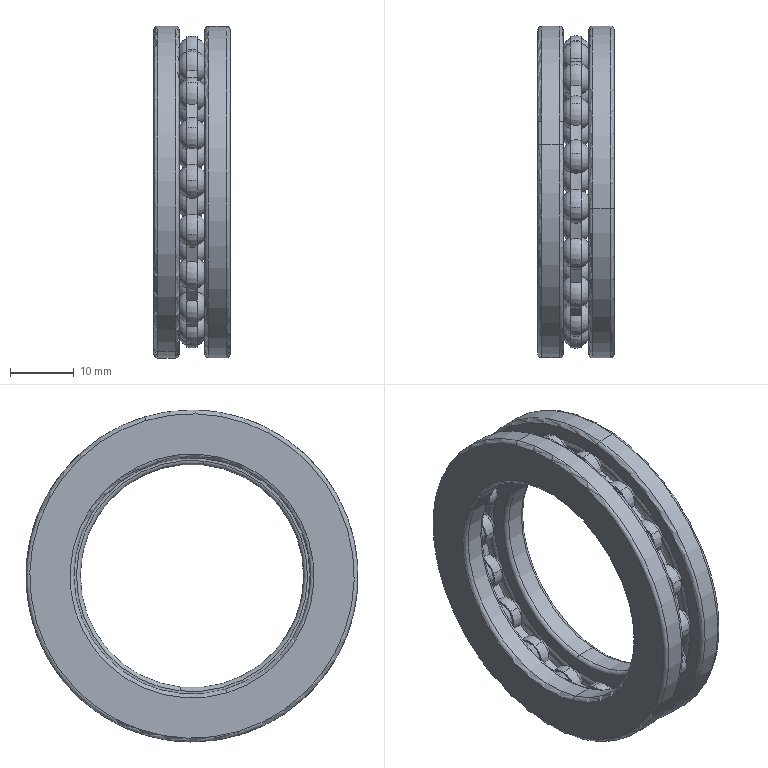Component | SolidWorks | 2-10-10WorkpieceAxisAssembly-1_2-10-9Bearing51107-1 | 21 solids | 224 faces | volume 9902 mm3 | sphere 144 | cylinder 44 | torus 28 | plane 8 | commonest cylinder face diameters 45.167 x18 41.833 x18 52 x4 35 x2 37 x2